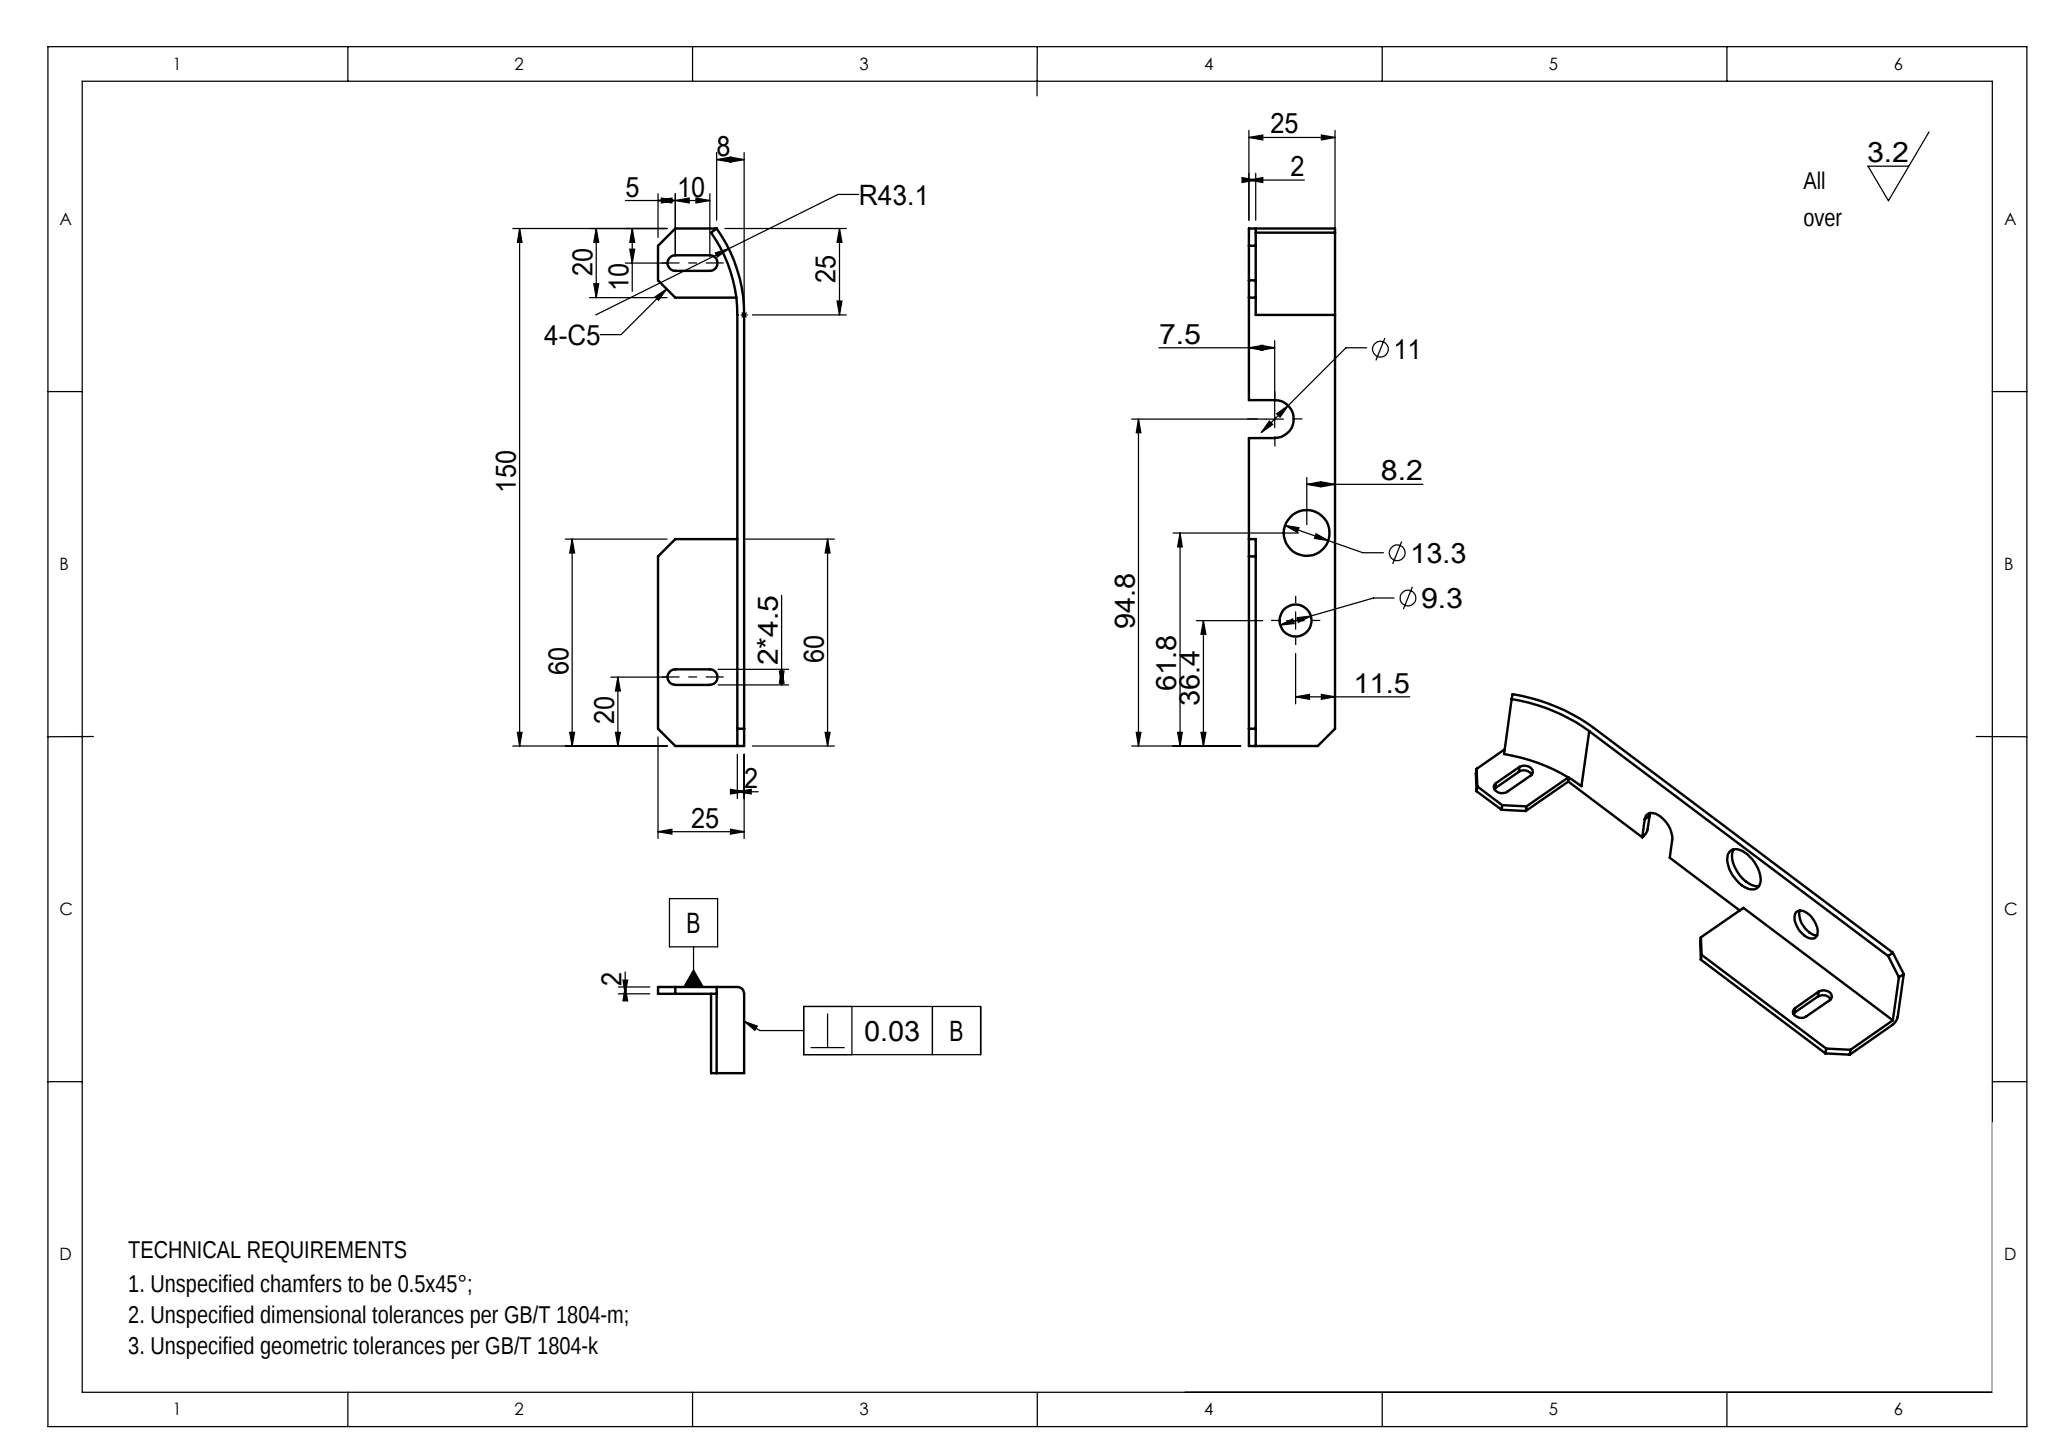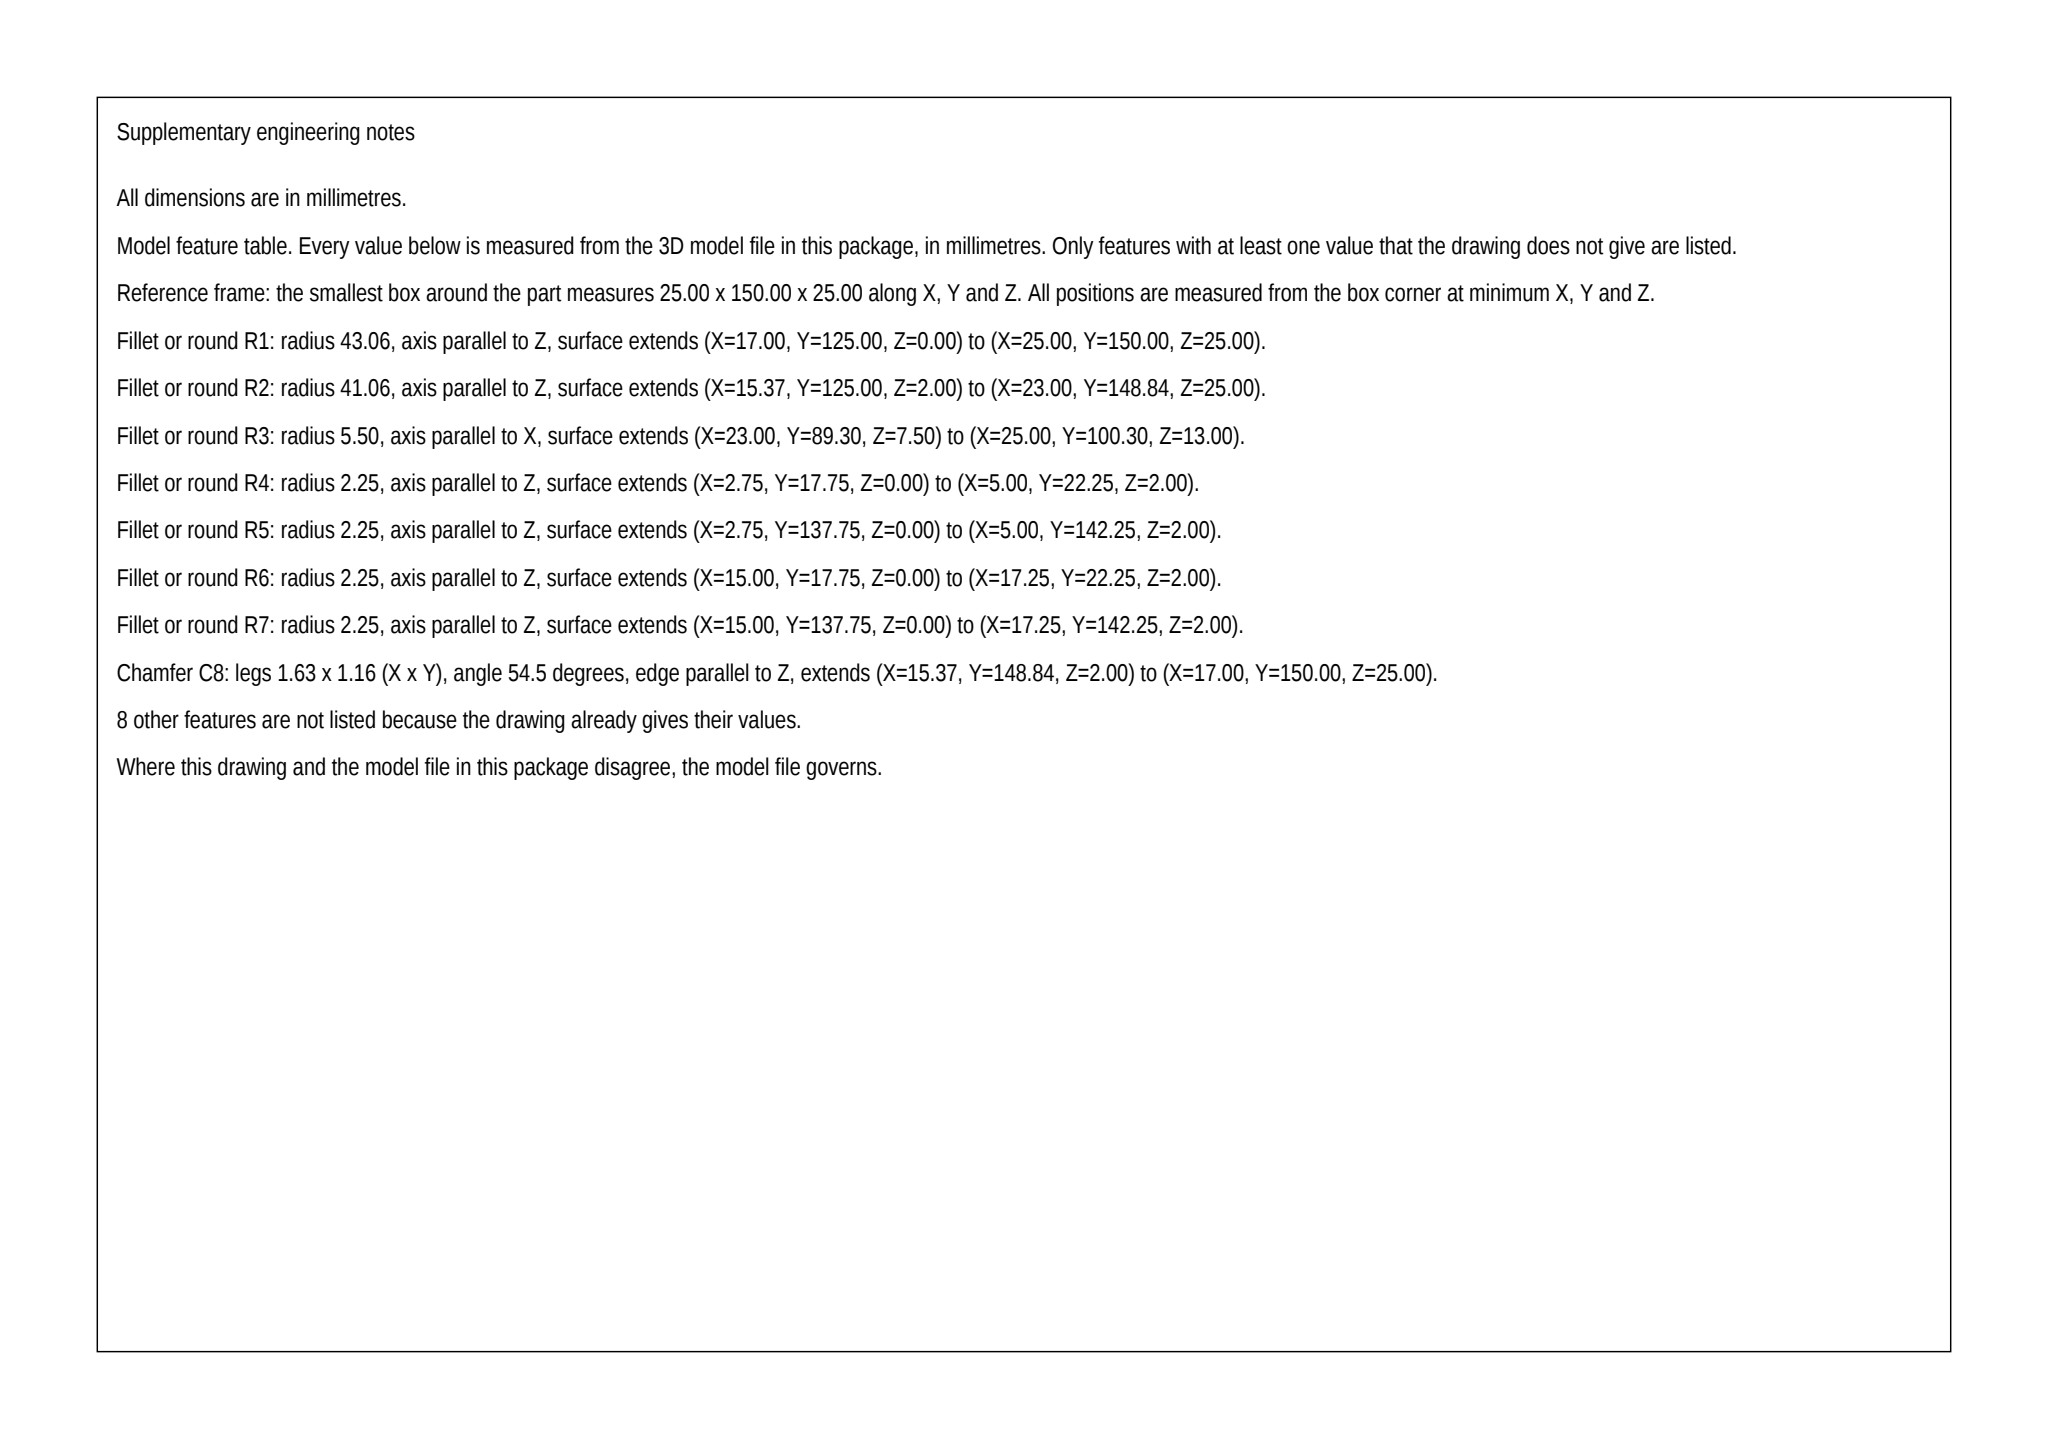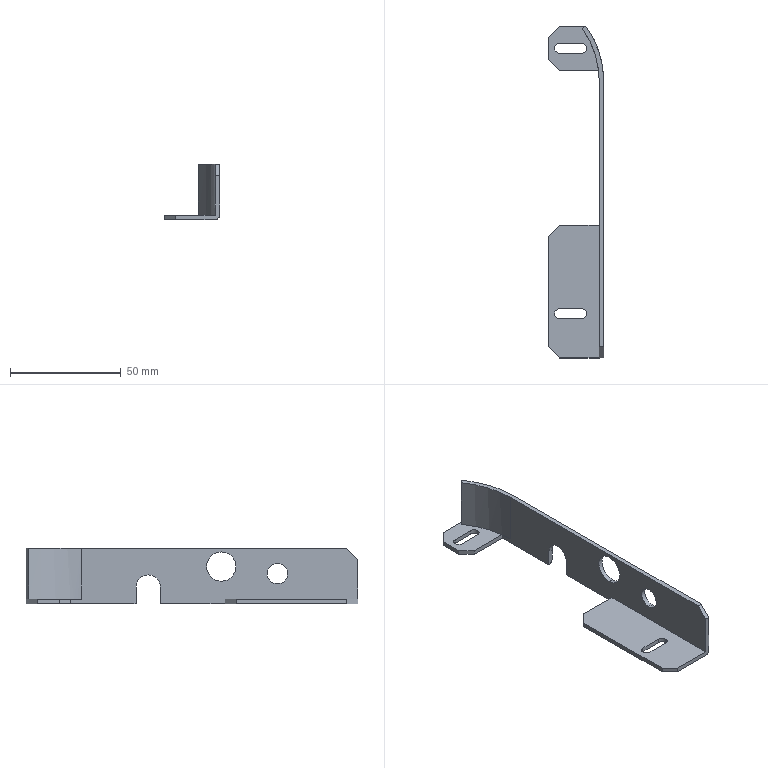Part | SolidWorks | mm | 1 solid | 42 faces | box 25 x 150 x 25 mm | volume 9957 mm3 | plane 26 | cylinder 16 | commonest cylinder face diameters 4.5 x6 9.269 x2 13.291 x2 11 x2 4 x2 82.125 x1 86.125 x1